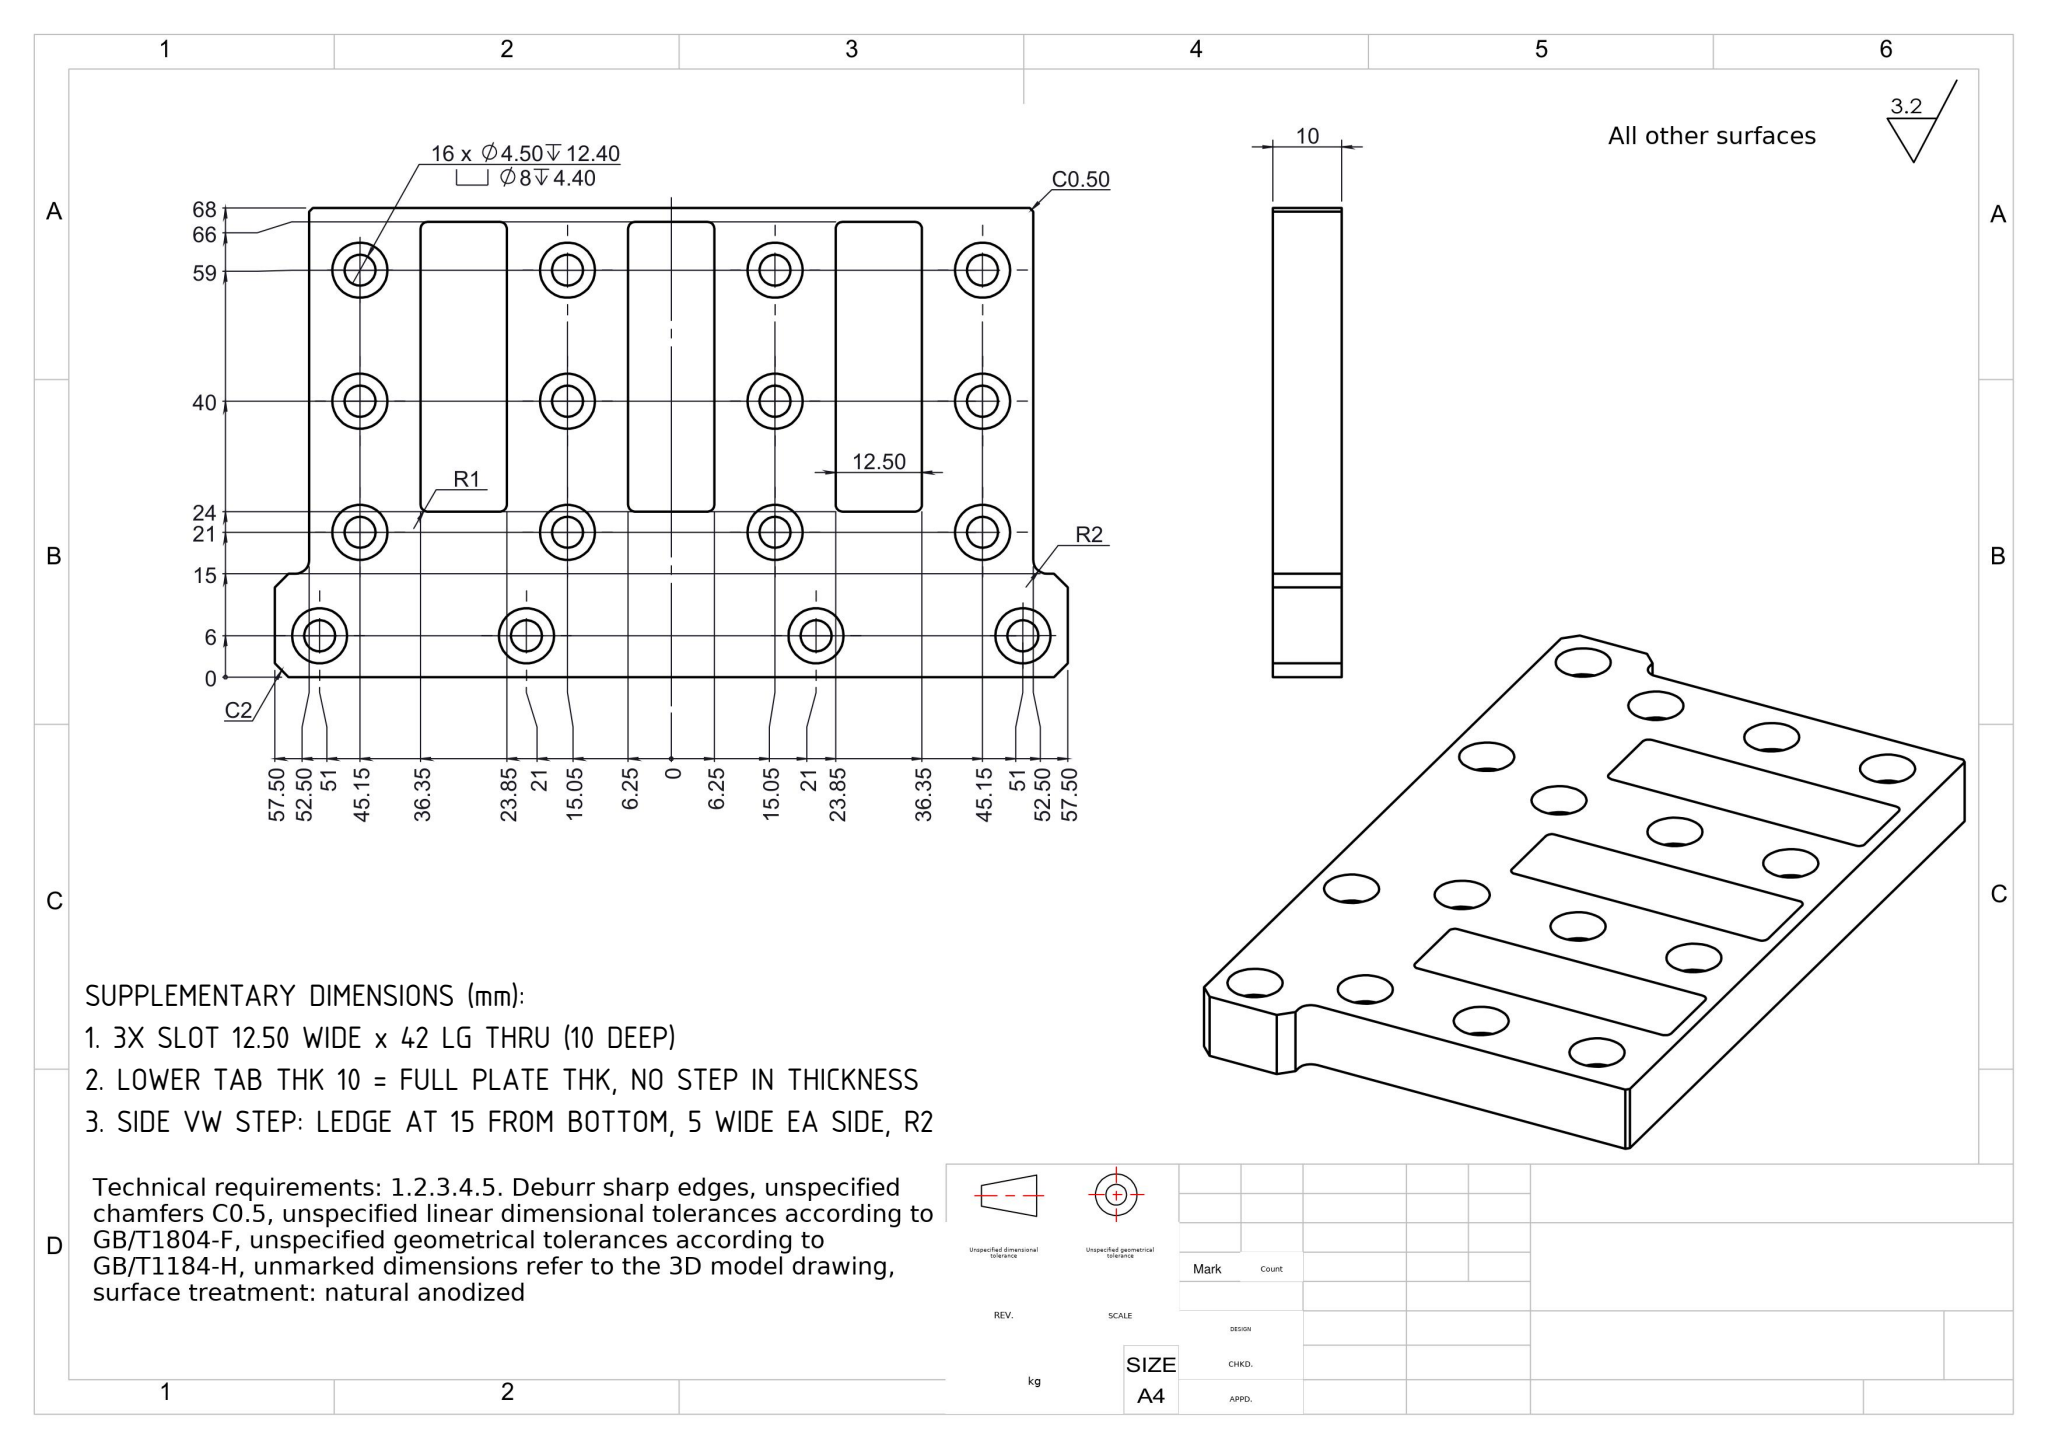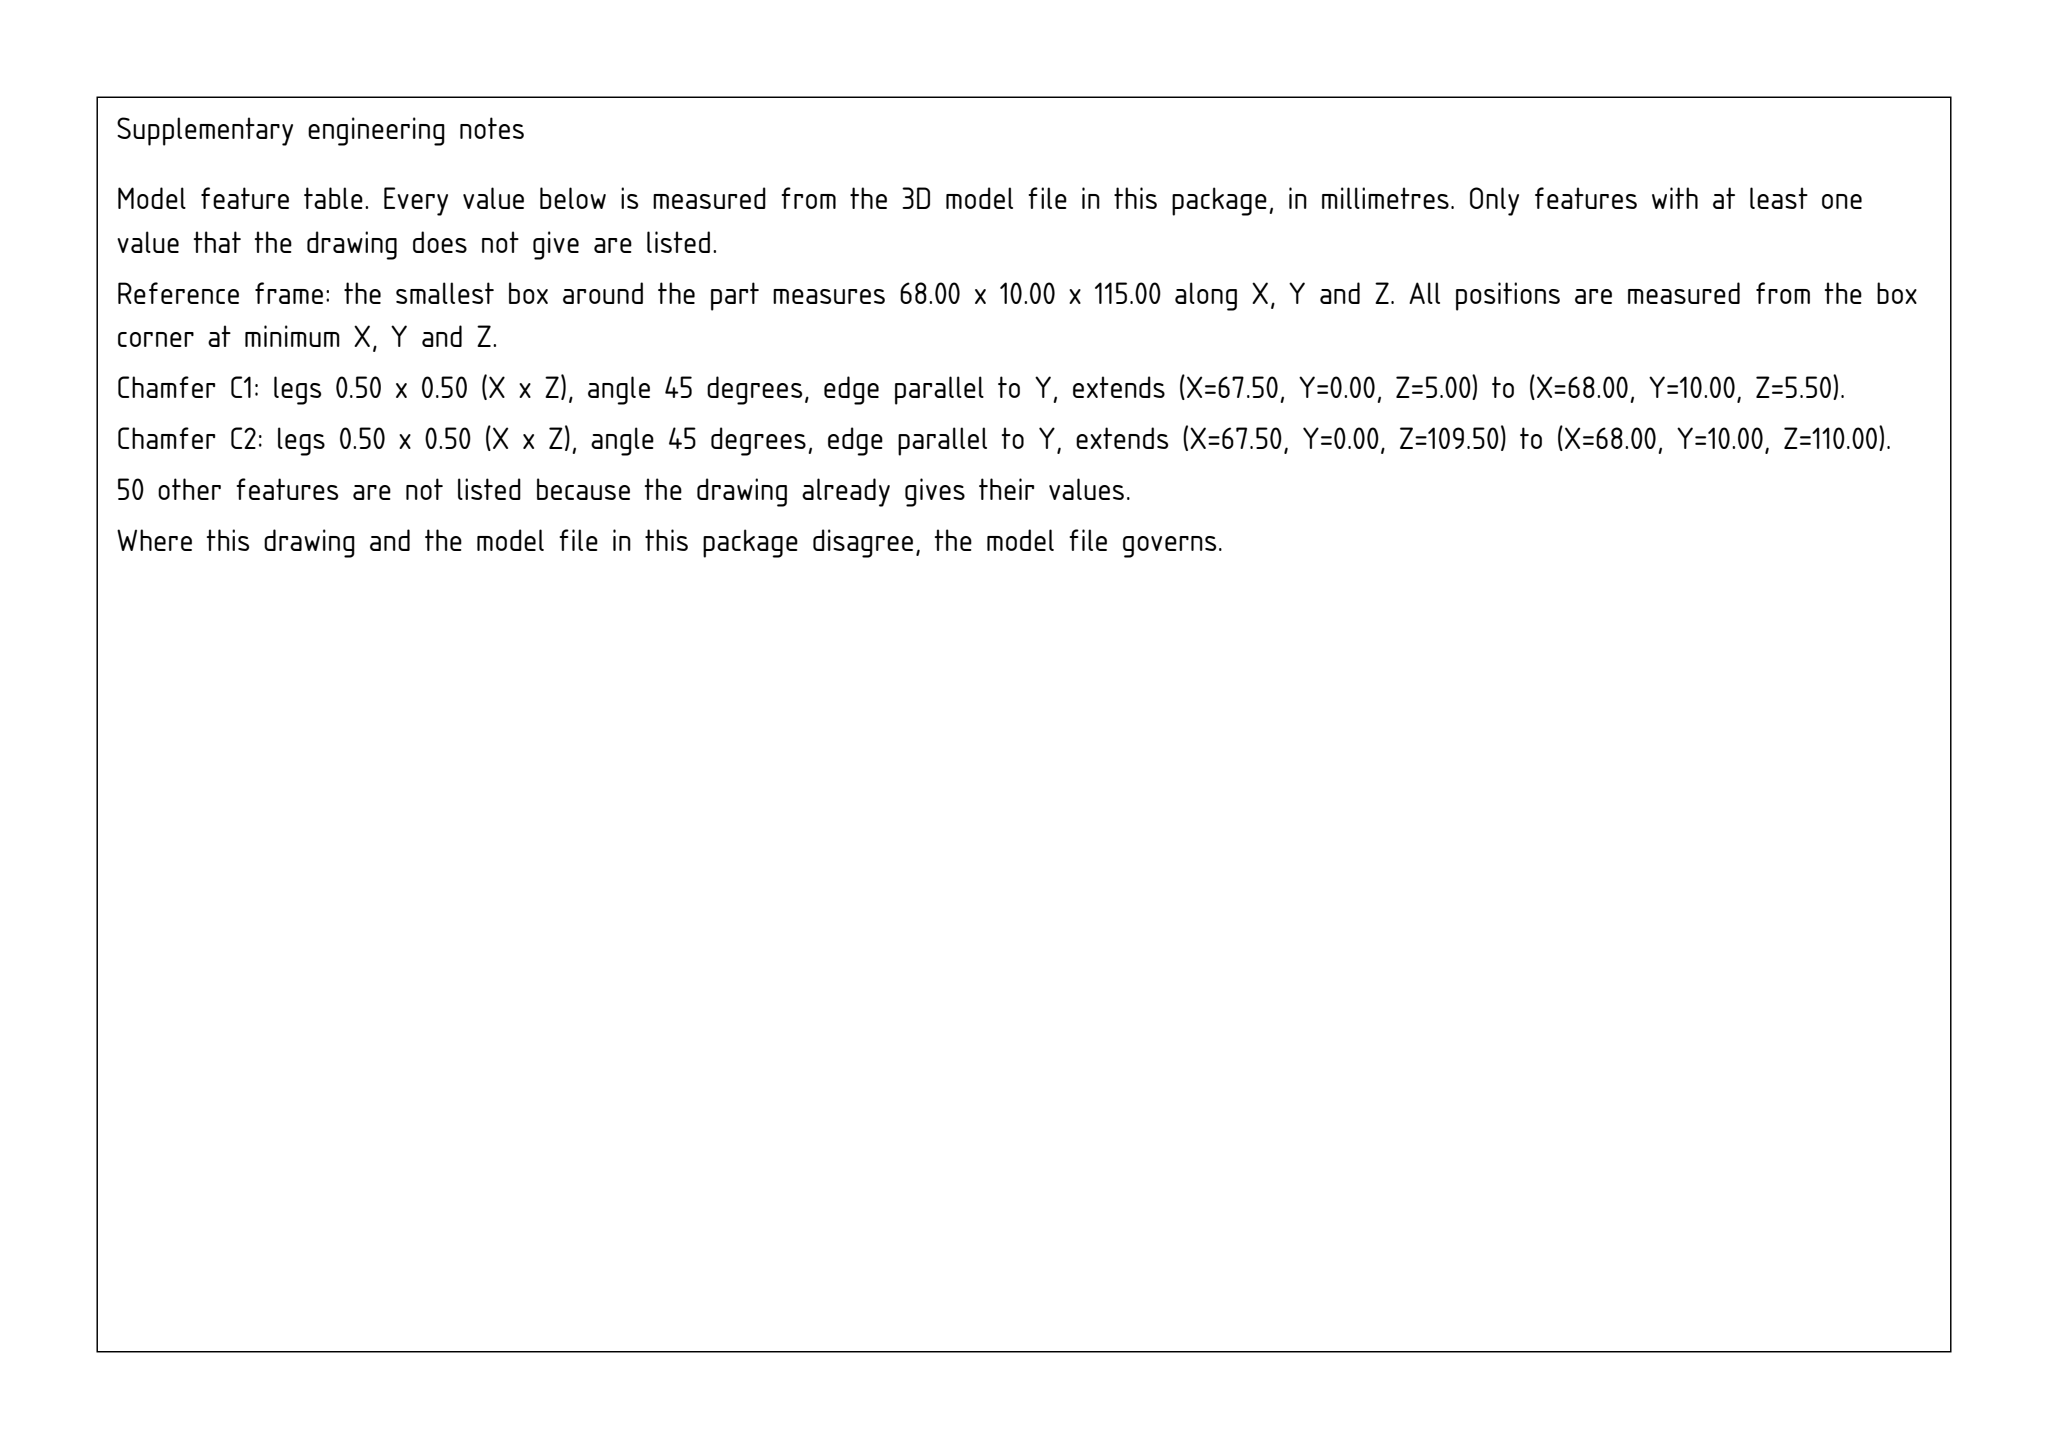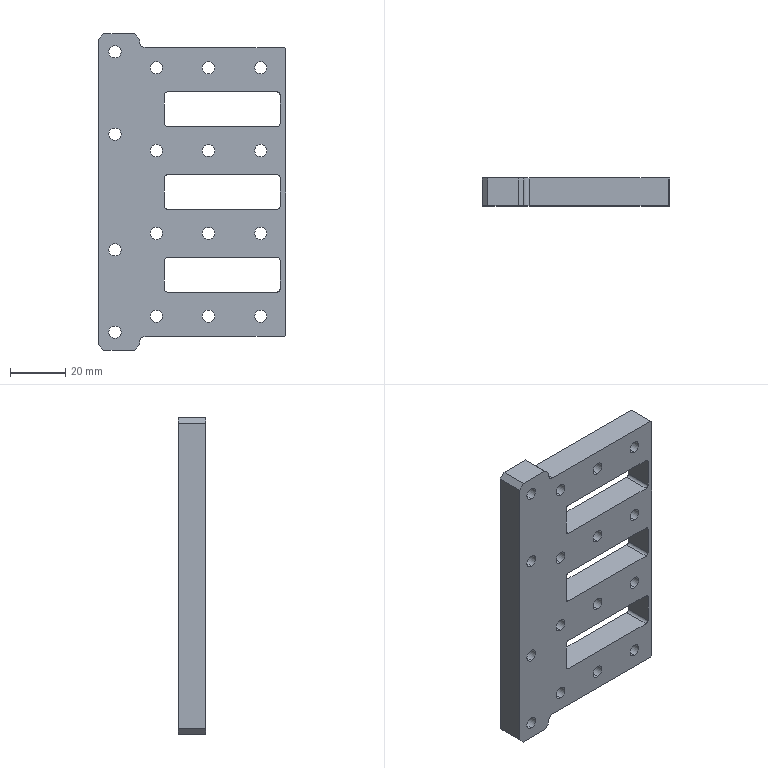Part | SolidWorks | mm | 1 solid | 122 faces | box 68 x 10 x 115 mm | volume 52147 mm3 | cylinder 78 | plane 44 | commonest cylinder face diameters 8 x32 4.5 x32 2 x12 4 x2
build123d program:
from build123d import *

# Parameters (mm, degrees)
SKETCH2_W                                       = 68
SKETCH2_H                                       = 115
BOSS_EXTRUDE1_DEPTH                             = 5
CUT_EXTRUDE3_DEPTH                              = 20
M4_HEX_SOCKET_HEAD_CAP_SCREW_CBORE1_D           = 4.5
M4_HEX_SOCKET_HEAD_CAP_SCREW_CBORE1_DEPTH       = 12.4
M4_HEX_SOCKET_HEAD_CAP_SCREW_CBORE1_CBORE_D     = 8
M4_HEX_SOCKET_HEAD_CAP_SCREW_CBORE1_CBORE_DEPTH = 4.4
M4_HEX_SOCKET_HEAD_CAP_SCREW_CBORE1_TIP         = 1.352
CHAMFER1_SIZE                                   = 2
SKETCH11_W                                      = 53
SKETCH11_H                                      = 5
CUT_EXTRUDE4_DEPTH                              = 68.544
CHAMFER2_SIZE                                   = 2
CHAMFER3_SIZE                                   = 0.5
FILLET1_R                                       = 2


with BuildPart() as part:
    # Sketch2 → Boss-Extrude1 (new, symmetric)
    with BuildSketch(Plane(origin=(0, 0, 0), x_dir=(1, 0, 0), z_dir=(0, 1, 0))):
        Rectangle(SKETCH2_W, SKETCH2_H)
    extrude(amount=BOSS_EXTRUDE1_DEPTH, both=True)

    # Sketch5 → Cut-Extrude3 (cut)
    with BuildSketch(Plane.XZ.offset(5)):
        with BuildLine():
            Line((31, -23.85), (-9, -23.85))
            ThreePointArc((-9, -23.85), (-9.707, -24.143), (-10, -24.85))
            Line((-10, -24.85), (-10, -35.35))
            ThreePointArc((-10, -35.35), (-9.707, -36.057), (-9, -36.35))
            Line((-9, -36.35), (31, -36.35))
            ThreePointArc((31, -36.35), (31.707, -36.057), (32, -35.35))
            Line((32, -35.35), (32, -24.85))
            ThreePointArc((32, -24.85), (31.707, -24.143), (31, -23.85))
        make_face()
        with BuildLine():
            Line((31, 6.25), (-9, 6.25))
            ThreePointArc((-9, 6.25), (-9.707, 5.957), (-10, 5.25))
            Line((-10, 5.25), (-10, -5.25))
            ThreePointArc((-10, -5.25), (-9.707, -5.957), (-9, -6.25))
            Line((-9, -6.25), (31, -6.25))
            ThreePointArc((31, -6.25), (31.707, -5.957), (32, -5.25))
            Line((32, -5.25), (32, 5.25))
            ThreePointArc((32, 5.25), (31.707, 5.957), (31, 6.25))
        make_face()
        with BuildLine():
            Line((31, 36.35), (-9, 36.35))
            ThreePointArc((-9, 36.35), (-9.707, 36.057), (-10, 35.35))
            Line((-10, 35.35), (-10, 24.85))
            ThreePointArc((-10, 24.85), (-9.707, 24.143), (-9, 23.85))
            Line((-9, 23.85), (31, 23.85))
            ThreePointArc((31, 23.85), (31.707, 24.143), (32, 24.85))
            Line((32, 24.85), (32, 35.35))
            ThreePointArc((32, 35.35), (31.707, 36.057), (31, 36.35))
        make_face()
    extrude(amount=-CUT_EXTRUDE3_DEPTH, mode=Mode.SUBTRACT)

    # M4 Hex Socket Head Cap Screw CBORE1
    with Locations(Plane(origin=(0, 5, 0), x_dir=(1, 0, 0), z_dir=(0, 1, 0))):
        with Locations((6, 45.15), (25, 45.15), (-13, 45.15), (-28, 51), (-13, 15.05), (6, 15.05), (25, 15.05), (-28, 21), (-13, -15.05), (6, -15.05), (25, -15.05), (6, -45.15), (25, -45.15), (-13, -45.15), (-28, -21), (-28, -51)):
            CounterBoreHole(M4_HEX_SOCKET_HEAD_CAP_SCREW_CBORE1_D / 2, M4_HEX_SOCKET_HEAD_CAP_SCREW_CBORE1_CBORE_D / 2, M4_HEX_SOCKET_HEAD_CAP_SCREW_CBORE1_CBORE_DEPTH, depth=M4_HEX_SOCKET_HEAD_CAP_SCREW_CBORE1_DEPTH)
            with Locations((0, 0, -(M4_HEX_SOCKET_HEAD_CAP_SCREW_CBORE1_DEPTH + M4_HEX_SOCKET_HEAD_CAP_SCREW_CBORE1_TIP / 2))):  # 118° drill point
                Cone(0, M4_HEX_SOCKET_HEAD_CAP_SCREW_CBORE1_D / 2, M4_HEX_SOCKET_HEAD_CAP_SCREW_CBORE1_TIP, mode=Mode.SUBTRACT)

    # Chamfer1
    chamfer1_edges = [part.edges().sort_by_distance(p)[0] for p in [
        (-34, 0, 57.5),
        (-34, 0, -57.5),
    ]]
    chamfer(chamfer1_edges, length=CHAMFER1_SIZE)

    # Sketch11 → Cut-Extrude4 (cut, through all)
    with BuildSketch(Plane.XZ.offset(5)):
        with Locations((7.5, 55)):
            Rectangle(SKETCH11_W, SKETCH11_H)
        with Locations((7.5, -55)):
            Rectangle(SKETCH11_W, SKETCH11_H)
    extrude(amount=-CUT_EXTRUDE4_DEPTH, mode=Mode.SUBTRACT)

    # Chamfer2
    chamfer2_edges = [part.edges().sort_by_distance(p)[0] for p in [
        (-19, 0, 57.5),
        (-19, 0, -57.5),
    ]]
    chamfer(chamfer2_edges, length=CHAMFER2_SIZE)

    # Chamfer3
    chamfer3_edges = [part.edges().sort_by_distance(p)[0] for p in [
        (34, 0, 52.5),
        (34, 0, -52.5),
    ]]
    chamfer(chamfer3_edges, length=CHAMFER3_SIZE)

    # Fillet1
    fillet1_edges = [part.edges().sort_by_distance(p)[0] for p in [
        (-19, 0, 52.5),
        (-19, 0, -52.5),
    ]]
    fillet(fillet1_edges, radius=FILLET1_R)


solid = part.part